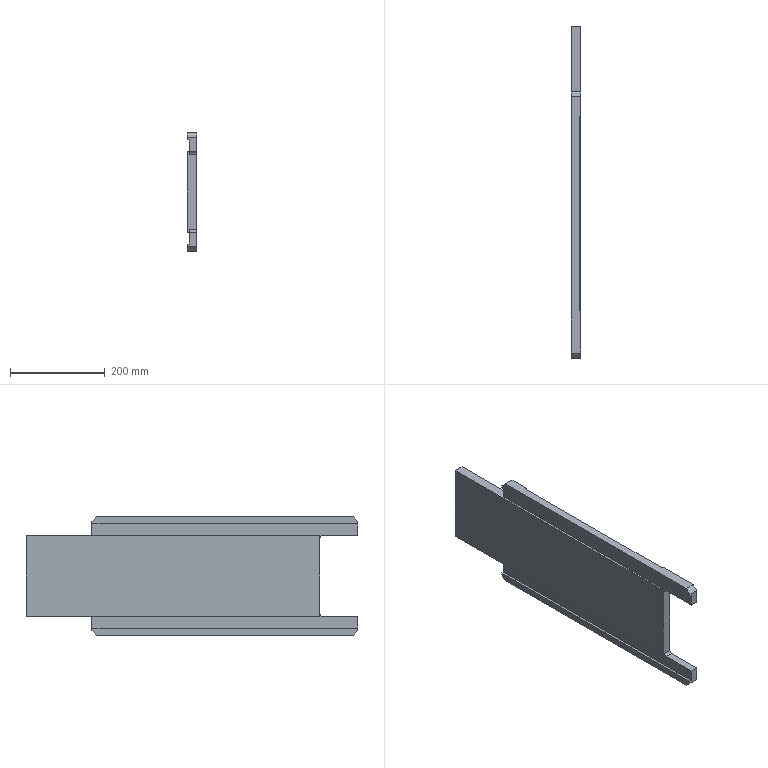Component | SolidWorks | 100-06-1 | 1 solid | 96 faces | box 20 x 700 x 250 mm | volume 2752383 mm3 | cylinder 36 | plane 32 | cone 28 | commonest cylinder face diameters 4.2 x28 6 x6 10 x2 | material 45
build123d program:
from build123d import *

# Parameters (mm, degrees)
SKETCH1_W             = 250
SKETCH1_H             = 700
BOSS_EXTRUDE1_DEPTH   = 10
SKETCH2_W             = 40
SKETCH2_H             = 139
CUT_EXTRUDE1_DEPTH    = 373.189
SKETCH3_W             = 55
SKETCH3_H             = 408
CUT_EXTRUDE2_DEPTH    = 3
M5_TAPPED_HOLE1_D     = 4.2
M5_TAPPED_HOLE1_DEPTH = 12.4
M5_TAPPED_HOLE1_TIP   = 1.262
SKETCH10_W            = 25
SKETCH10_H            = 561
CUT_EXTRUDE5_DEPTH    = 4
SKETCH12_R            = 3
CUT_EXTRUDE7_DEPTH    = 3
SKETCH13_W            = 170
SKETCH13_H            = 80
CUT_EXTRUDE8_DEPTH    = 373.189
CHAMFER1_SIZE         = 10
FILLET1_R             = 5


with BuildPart() as part:
    # Sketch1 → Boss-Extrude1 (new, symmetric)
    with BuildSketch(Plane(origin=(0, 0, 0), x_dir=(1, 0, 0), z_dir=(0, 1, 0))):
        Rectangle(SKETCH1_W, SKETCH1_H)
    extrude(amount=BOSS_EXTRUDE1_DEPTH, both=True)

    # Sketch2 → Cut-Extrude1 (cut, through all)
    with BuildSketch(Plane(origin=(0, 10, 0), x_dir=(1, 0, 0), z_dir=(0, 1, 0))):
        with Locations((-105, 280.5)):
            Rectangle(SKETCH2_W, SKETCH2_H)
        with Locations((105, 280.5)):
            Rectangle(SKETCH2_W, SKETCH2_H)
    extrude(amount=-CUT_EXTRUDE1_DEPTH, mode=Mode.SUBTRACT)

    # Sketch3 → Cut-Extrude2 (cut)
    with BuildSketch(Plane(origin=(0, 10, 0), x_dir=(1, 0, 0), z_dir=(0, 1, 0))):
        with Locations((-97.5, -46)):
            Rectangle(SKETCH3_W, SKETCH3_H)
        with Locations((97.5, -46)):
            Rectangle(SKETCH3_W, SKETCH3_H)
    extrude(amount=-CUT_EXTRUDE2_DEPTH, mode=Mode.SUBTRACT)

    # M5 Tapped Hole1
    with Locations(Plane(origin=(0, 7, 0), x_dir=(1, 0, 0), z_dir=(0, 1, 0))):
        with Locations((-80, -45.5), (-80, 14.5), (-80, 74.5), (-80, 134.5), (-80, -105.5), (-80, -165.5), (-80, -225.5), (80, 134.5), (80, 74.5), (80, 14.5), (80, -45.5), (80, -105.5), (80, -165.5), (80, -225.5)):
            Hole(M5_TAPPED_HOLE1_D / 2, depth=M5_TAPPED_HOLE1_DEPTH)
            with Locations((0, 0, -(M5_TAPPED_HOLE1_DEPTH + M5_TAPPED_HOLE1_TIP / 2))):  # 118° drill point
                Cone(0, M5_TAPPED_HOLE1_D / 2, M5_TAPPED_HOLE1_TIP, mode=Mode.SUBTRACT)

    # Sketch10 → Cut-Extrude5 (cut)
    with BuildSketch(Plane.XZ.offset(10)):
        with Locations((-97.5, 69.5)):
            Rectangle(SKETCH10_W, SKETCH10_H)
    cut_extrude5 = extrude(amount=-CUT_EXTRUDE5_DEPTH, mode=Mode.SUBTRACT)

    # Mirror2: Cut-Extrude5 across plane
    add(cut_extrude5.mirror(Plane(origin=(0, 0, 0), x_dir=(0, 0, 1), z_dir=(1, 0, 0))), mode=Mode.SUBTRACT)

    # Sketch12 → Cut-Extrude7 (cut)
    with BuildSketch(Plane(origin=(0, 10, 0), x_dir=(1, 0, 0), z_dir=(0, 1, 0))):
        with Locations((-72.12, 155.88)):
            Circle(SKETCH12_R)
        with Locations((-72.12, -247.88)):
            Circle(SKETCH12_R)
        with Locations((72.12, -247.88)):
            Circle(SKETCH12_R)
        with Locations((72.12, 155.88)):
            Circle(SKETCH12_R)
    extrude(amount=-CUT_EXTRUDE7_DEPTH, mode=Mode.SUBTRACT)

    # Sketch13 → Cut-Extrude8 (cut, through all)
    with BuildSketch(Plane(origin=(0, 10, 0), x_dir=(1, 0, 0), z_dir=(0, 1, 0))):
        with Locations((0, -310)):
            Rectangle(SKETCH13_W, SKETCH13_H)
    extrude(amount=-CUT_EXTRUDE8_DEPTH, mode=Mode.SUBTRACT)

    # Chamfer1
    chamfer1_edges = [part.edges().sort_by_distance(p)[0] for p in [
        (-125, 0, -211),
        (125, 0, -211),
        (125, 0, 350),
        (-125, 0, 350),
    ]]
    chamfer(chamfer1_edges, length=CHAMFER1_SIZE)

    # Fillet1
    fillet1_edges = [part.edges().sort_by_distance(p)[0] for p in [
        (85, 2, 270),
        (-85, 2, 270),
    ]]
    fillet(fillet1_edges, radius=FILLET1_R)


solid = part.part

# Placed as in the assembly
solid = solid.moved(Location((56, 490, 0), (90, 0, -90)))